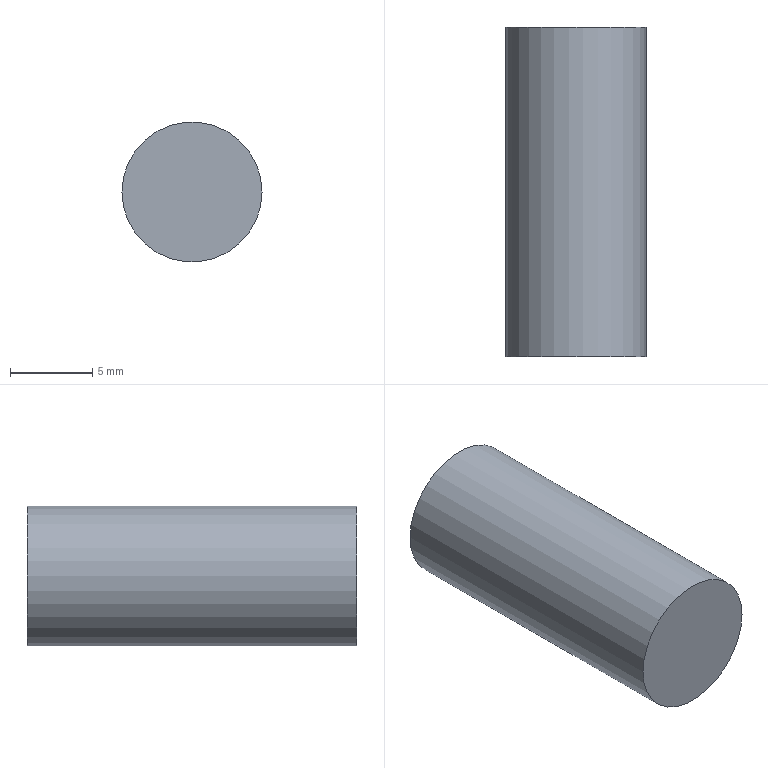Component | NX | SCREW_1_2 | 1 solid | 3 faces | box 8.5 x 20 x 8.5 mm | volume 1135 mm3 | plane 2 | cylinder 1 | commonest cylinder face diameters 8.5 x1
STEP:
#1=CARTESIAN_POINT('',(0.,0.,0.));
#2=DIRECTION('',(0.,0.,1.));
#3=DIRECTION('',(1.,0.,0.));
#4=AXIS2_PLACEMENT_3D('',#1,#2,#3);
#5=CARTESIAN_POINT('',(4.25,160.,41.));
#6=VERTEX_POINT('',#5);
#7=CARTESIAN_POINT('',(0.,160.,41.));
#8=DIRECTION('',(0.,1.,0.));
#9=DIRECTION('',(1.,0.,0.));
#10=AXIS2_PLACEMENT_3D('',#7,#8,#9);
#11=CIRCLE('',#10,4.25);
#12=CARTESIAN_POINT('',(0.,160.,41.));
#13=DIRECTION('',(0.,-1.,0.));
#14=DIRECTION('',(1.,0.,0.));
#15=AXIS2_PLACEMENT_3D('',#12,#13,#14);
#16=CYLINDRICAL_SURFACE('',#15,4.25);
#17=CARTESIAN_POINT('',(6.283,0.));
#18=DIRECTION('',(-1.,0.));
#19=VECTOR('',#18,1.);
#20=LINE('',#17,#19);
#21=(GEOMETRIC_REPRESENTATION_CONTEXT(2)PARAMETRIC_REPRESENTATION_CONTEXT()REPRESENTATION_CONTEXT('',''));
#22=DEFINITIONAL_REPRESENTATION('',(#20),#21);
#23=PCURVE('',#16,#22);
#24=CARTESIAN_POINT('',(0.,160.,41.));
#25=DIRECTION('',(0.,1.,0.));
#26=DIRECTION('',(-1.,0.,0.));
#27=AXIS2_PLACEMENT_3D('',#24,#25,#26);
#28=PLANE('',#27);
#29=CARTESIAN_POINT('',(0.,0.));
#30=DIRECTION('',(-1.,0.));
#31=AXIS2_PLACEMENT_2D('',#29,#30);
#32=CIRCLE('',#31,4.25);
#33=(GEOMETRIC_REPRESENTATION_CONTEXT(2)PARAMETRIC_REPRESENTATION_CONTEXT()REPRESENTATION_CONTEXT('',''));
#34=DEFINITIONAL_REPRESENTATION('',(#32),#33);
#35=PCURVE('',#28,#34);
#36=SURFACE_CURVE('',#11,(#23,#35),.PCURVE_S1.);
#37=EDGE_CURVE('',#6,#6,#36,.T.);
#38=ORIENTED_EDGE('',*,*,#37,.F.);
#39=CARTESIAN_POINT('',(4.25,140.,41.));
#40=VERTEX_POINT('',#39);
#41=CARTESIAN_POINT('',(4.25,160.,41.));
#42=CARTESIAN_POINT('',(4.25,140.,41.));
#43=B_SPLINE_CURVE_WITH_KNOTS('',1,(#41,#42),.UNSPECIFIED.,.F.,.F.,(2,2),(0.,20.),.PIECEWISE_BEZIER_KNOTS.);
#44=CARTESIAN_POINT('',(6.283,0.));
#45=DIRECTION('',(0.,1.));
#46=VECTOR('',#45,1.);
#47=LINE('',#44,#46);
#48=(GEOMETRIC_REPRESENTATION_CONTEXT(2)PARAMETRIC_REPRESENTATION_CONTEXT()REPRESENTATION_CONTEXT('',''));
#49=DEFINITIONAL_REPRESENTATION('',(#47),#48);
#50=PCURVE('',#16,#49);
#51=CARTESIAN_POINT('',(0.,0.));
#52=DIRECTION('',(0.,1.));
#53=VECTOR('',#52,1.);
#54=LINE('',#51,#53);
#55=(GEOMETRIC_REPRESENTATION_CONTEXT(2)PARAMETRIC_REPRESENTATION_CONTEXT()REPRESENTATION_CONTEXT('',''));
#56=DEFINITIONAL_REPRESENTATION('',(#54),#55);
#57=PCURVE('',#16,#56);
#58=SEAM_CURVE('',#43,(#50,#57),.PCURVE_S1.);
#59=EDGE_CURVE('',#6,#40,#58,.T.);
#60=ORIENTED_EDGE('',*,*,#59,.T.);
#61=CARTESIAN_POINT('',(0.,140.,41.));
#62=DIRECTION('',(0.,1.,0.));
#63=DIRECTION('',(1.,0.,0.));
#64=AXIS2_PLACEMENT_3D('',#61,#62,#63);
#65=CIRCLE('',#64,4.25);
#66=CARTESIAN_POINT('',(6.283,20.));
#67=DIRECTION('',(-1.,0.));
#68=VECTOR('',#67,1.);
#69=LINE('',#66,#68);
#70=(GEOMETRIC_REPRESENTATION_CONTEXT(2)PARAMETRIC_REPRESENTATION_CONTEXT()REPRESENTATION_CONTEXT('',''));
#71=DEFINITIONAL_REPRESENTATION('',(#69),#70);
#72=PCURVE('',#16,#71);
#73=CARTESIAN_POINT('',(0.,140.,41.));
#74=DIRECTION('',(0.,1.,0.));
#75=DIRECTION('',(-1.,0.,0.));
#76=AXIS2_PLACEMENT_3D('',#73,#74,#75);
#77=PLANE('',#76);
#78=CARTESIAN_POINT('',(0.,0.));
#79=DIRECTION('',(-1.,0.));
#80=AXIS2_PLACEMENT_2D('',#78,#79);
#81=CIRCLE('',#80,4.25);
#82=(GEOMETRIC_REPRESENTATION_CONTEXT(2)PARAMETRIC_REPRESENTATION_CONTEXT()REPRESENTATION_CONTEXT('',''));
#83=DEFINITIONAL_REPRESENTATION('',(#81),#82);
#84=PCURVE('',#77,#83);
#85=SURFACE_CURVE('',#65,(#72,#84),.PCURVE_S1.);
#86=EDGE_CURVE('',#40,#40,#85,.T.);
#87=ORIENTED_EDGE('',*,*,#86,.T.);
#88=ORIENTED_EDGE('',*,*,#59,.F.);
#89=EDGE_LOOP('',(#38,#60,#87,#88));
#90=FACE_BOUND('',#89,.T.);
#91=ADVANCED_FACE('',(#90),#16,.T.);
#92=ORIENTED_EDGE('',*,*,#37,.T.);
#93=EDGE_LOOP('',(#92));
#94=FACE_BOUND('',#93,.T.);
#95=ADVANCED_FACE('',(#94),#28,.T.);
#96=ORIENTED_EDGE('',*,*,#86,.F.);
#97=EDGE_LOOP('',(#96));
#98=FACE_BOUND('',#97,.T.);
#99=ADVANCED_FACE('',(#98),#77,.F.);
#100=CLOSED_SHELL('',(#91,#95,#99));
#101=MANIFOLD_SOLID_BREP('',#100);
#102=(LENGTH_UNIT()NAMED_UNIT(*)SI_UNIT(.MILLI.,.METRE.));
#103=UNCERTAINTY_MEASURE_WITH_UNIT(LENGTH_MEASURE(0.00001),#102,'','');
#104=(NAMED_UNIT(*)PLANE_ANGLE_UNIT()SI_UNIT($,.RADIAN.));
#105=(NAMED_UNIT(*)SI_UNIT($,.STERADIAN.)SOLID_ANGLE_UNIT());
#106=(GEOMETRIC_REPRESENTATION_CONTEXT(3)GLOBAL_UNCERTAINTY_ASSIGNED_CONTEXT((#103))GLOBAL_UNIT_ASSIGNED_CONTEXT((#102,#104,#105))REPRESENTATION_CONTEXT('',''));
#107=ADVANCED_BREP_SHAPE_REPRESENTATION('',(#4,#101),#106);